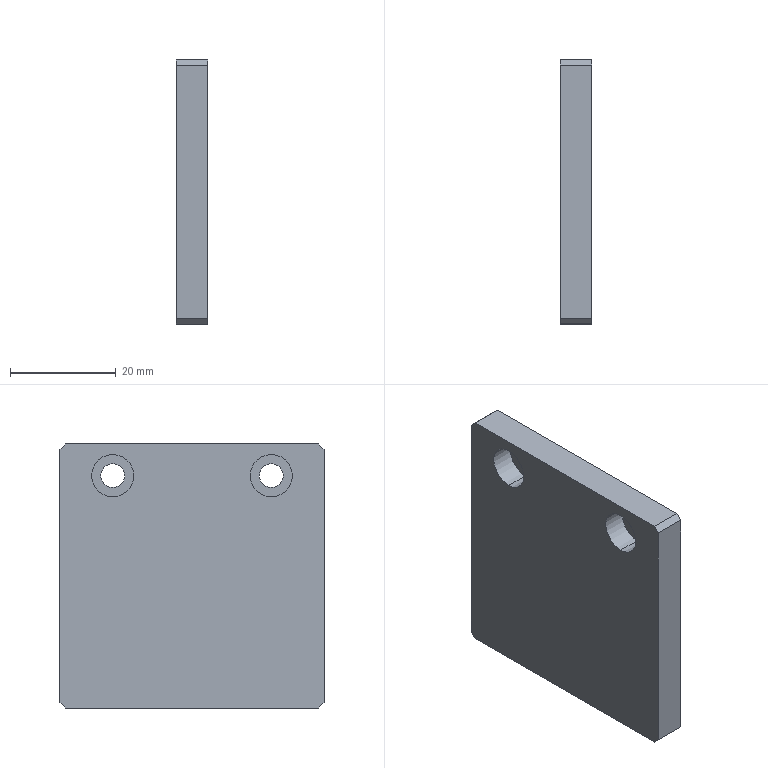Component | SolidWorks | 002MaterialPickingModuleA-1_J-008-1 | 1 solid | 20 faces | box 6 x 50 x 50 mm | volume 14495 mm3 | plane 12 | cylinder 8 | commonest cylinder face diameters 8 x4 4.5 x4 | material 45
build123d program:
from build123d import *

# Parameters (mm, degrees)
SKETCH1_W                                       = 50
SKETCH1_H                                       = 50
BOSS_EXTRUDE1_DEPTH                             = 6
M4_HEX_SOCKET_HEAD_CAP_SCREW_CBORE1_D           = 4.5
M4_HEX_SOCKET_HEAD_CAP_SCREW_CBORE1_CBORE_D     = 8
M4_HEX_SOCKET_HEAD_CAP_SCREW_CBORE1_CBORE_DEPTH = 4.4
CHAMFER1_SIZE                                   = 1


with BuildPart() as part:
    # Sketch1 → Boss-Extrude1 (new body)
    with BuildSketch(Plane(origin=(0, 0, 0), x_dir=(0, 0, -1), z_dir=(1, 0, 0))):
        Rectangle(SKETCH1_W, SKETCH1_H)
    extrude(amount=BOSS_EXTRUDE1_DEPTH)

    # M4 Hex Socket Head Cap Screw CBORE1 (through all)
    with Locations(Plane.ZY):
        with Locations((-19, 15), (-19, -15)):
            CounterBoreHole(M4_HEX_SOCKET_HEAD_CAP_SCREW_CBORE1_D / 2, M4_HEX_SOCKET_HEAD_CAP_SCREW_CBORE1_CBORE_D / 2, M4_HEX_SOCKET_HEAD_CAP_SCREW_CBORE1_CBORE_DEPTH)

    # Chamfer1
    chamfer1_edges = [part.edges().sort_by_distance(p)[0] for p in [
        (3, 25, 25),
        (3, 25, -25),
        (3, -25, -25),
        (3, -25, 25),
    ]]
    chamfer(chamfer1_edges, length=CHAMFER1_SIZE)


solid = part.part

# Placed as in the assembly
solid = solid.moved(Location((-5.675, 326.019, 403.231), (180, 0, 0)))
STEP:
#1=COLOUR_RGB('',0.7922,0.8196,0.9333);
#2=FILL_AREA_STYLE_COLOUR('',#1);
#3=FILL_AREA_STYLE('',(#2));
#4=SURFACE_STYLE_FILL_AREA(#3);
#5=SURFACE_SIDE_STYLE('',(#4));
#6=SURFACE_STYLE_USAGE(.BOTH.,#5);
#7=PRESENTATION_STYLE_ASSIGNMENT((#6));
#8=CARTESIAN_POINT('',(-0.0502,12.245,16.781));
#9=VERTEX_POINT('',#8);
#10=CARTESIAN_POINT('',(-0.0502,12.245,16.466));
#11=VERTEX_POINT('',#10);
#12=CARTESIAN_POINT('',(-0.0502,12.245,16.623));
#13=DIRECTION('',(-1.,0.,0.));
#14=DIRECTION('',(0.,0.,-1.));
#15=AXIS2_PLACEMENT_3D('',#12,#13,#14);
#16=CIRCLE('',#15,0.1575);
#17=EDGE_CURVE('',#9,#11,#16,.T.);
#18=ORIENTED_EDGE('',*,*,#17,.F.);
#19=CARTESIAN_POINT('',(-0.2234,12.245,16.781));
#20=VERTEX_POINT('',#19);
#21=CARTESIAN_POINT('',(-0.2234,12.245,16.781));
#22=DIRECTION('',(-1.,0.,0.));
#23=VECTOR('',#22,39.37);
#24=LINE('',#21,#23);
#25=EDGE_CURVE('',#9,#20,#24,.T.);
#26=ORIENTED_EDGE('',*,*,#25,.T.);
#27=CARTESIAN_POINT('',(-0.2234,12.245,16.466));
#28=VERTEX_POINT('',#27);
#29=CARTESIAN_POINT('',(-0.2234,12.245,16.623));
#30=DIRECTION('',(-1.,0.,0.));
#31=DIRECTION('',(0.,0.,-1.));
#32=AXIS2_PLACEMENT_3D('',#29,#30,#31);
#33=CIRCLE('',#32,0.1575);
#34=EDGE_CURVE('',#20,#28,#33,.T.);
#35=ORIENTED_EDGE('',*,*,#34,.T.);
#36=CARTESIAN_POINT('',(-0.2234,12.245,16.466));
#37=DIRECTION('',(-1.,0.,0.));
#38=VECTOR('',#37,39.37);
#39=LINE('',#36,#38);
#40=EDGE_CURVE('',#11,#28,#39,.T.);
#41=ORIENTED_EDGE('',*,*,#40,.F.);
#42=EDGE_LOOP('',(#18,#26,#35,#41));
#43=FACE_OUTER_BOUND('',#42,.T.);
#44=CARTESIAN_POINT('',(-0.2234,12.245,16.623));
#45=DIRECTION('',(-1.,0.,0.));
#46=DIRECTION('',(0.,0.,-1.));
#47=AXIS2_PLACEMENT_3D('',#44,#45,#46);
#48=CYLINDRICAL_SURFACE('',#47,0.1575);
#49=ADVANCED_FACE('',(#43),#48,.F.);
#50=CARTESIAN_POINT('',(0.01279,12.245,16.712));
#51=VERTEX_POINT('',#50);
#52=CARTESIAN_POINT('',(0.01279,12.245,16.535));
#53=VERTEX_POINT('',#52);
#54=CARTESIAN_POINT('',(0.01279,12.245,16.623));
#55=DIRECTION('',(-1.,0.,0.));
#56=DIRECTION('',(0.,0.,-1.));
#57=AXIS2_PLACEMENT_3D('',#54,#55,#56);
#58=CIRCLE('',#57,0.08858);
#59=EDGE_CURVE('',#51,#53,#58,.T.);
#60=ORIENTED_EDGE('',*,*,#59,.F.);
#61=CARTESIAN_POINT('',(-0.0502,12.245,16.712));
#62=VERTEX_POINT('',#61);
#63=CARTESIAN_POINT('',(-0.2234,12.245,16.712));
#64=DIRECTION('',(-1.,0.,0.));
#65=VECTOR('',#64,39.37);
#66=LINE('',#63,#65);
#67=EDGE_CURVE('',#51,#62,#66,.T.);
#68=ORIENTED_EDGE('',*,*,#67,.T.);
#69=CARTESIAN_POINT('',(-0.0502,12.245,16.535));
#70=VERTEX_POINT('',#69);
#71=CARTESIAN_POINT('',(-0.0502,12.245,16.623));
#72=DIRECTION('',(-1.,0.,0.));
#73=DIRECTION('',(0.,0.,-1.));
#74=AXIS2_PLACEMENT_3D('',#71,#72,#73);
#75=CIRCLE('',#74,0.08858);
#76=EDGE_CURVE('',#62,#70,#75,.T.);
#77=ORIENTED_EDGE('',*,*,#76,.T.);
#78=CARTESIAN_POINT('',(-0.2234,12.245,16.535));
#79=DIRECTION('',(-1.,0.,0.));
#80=VECTOR('',#79,39.37);
#81=LINE('',#78,#80);
#82=EDGE_CURVE('',#53,#70,#81,.T.);
#83=ORIENTED_EDGE('',*,*,#82,.F.);
#84=EDGE_LOOP('',(#60,#68,#77,#83));
#85=FACE_OUTER_BOUND('',#84,.T.);
#86=CARTESIAN_POINT('',(-0.2234,12.245,16.623));
#87=DIRECTION('',(-1.,0.,0.));
#88=DIRECTION('',(0.,0.,-1.));
#89=AXIS2_PLACEMENT_3D('',#86,#87,#88);
#90=CYLINDRICAL_SURFACE('',#89,0.08858);
#91=ADVANCED_FACE('',(#85),#90,.F.);
#92=CARTESIAN_POINT('',(-0.0502,13.426,16.781));
#93=VERTEX_POINT('',#92);
#94=CARTESIAN_POINT('',(-0.0502,13.426,16.466));
#95=VERTEX_POINT('',#94);
#96=CARTESIAN_POINT('',(-0.0502,13.426,16.623));
#97=DIRECTION('',(-1.,0.,0.));
#98=DIRECTION('',(0.,0.,-1.));
#99=AXIS2_PLACEMENT_3D('',#96,#97,#98);
#100=CIRCLE('',#99,0.1575);
#101=EDGE_CURVE('',#93,#95,#100,.T.);
#102=ORIENTED_EDGE('',*,*,#101,.F.);
#103=CARTESIAN_POINT('',(-0.2234,13.426,16.781));
#104=VERTEX_POINT('',#103);
#105=CARTESIAN_POINT('',(-0.2234,13.426,16.781));
#106=DIRECTION('',(-1.,0.,0.));
#107=VECTOR('',#106,39.37);
#108=LINE('',#105,#107);
#109=EDGE_CURVE('',#93,#104,#108,.T.);
#110=ORIENTED_EDGE('',*,*,#109,.T.);
#111=CARTESIAN_POINT('',(-0.2234,13.426,16.466));
#112=VERTEX_POINT('',#111);
#113=CARTESIAN_POINT('',(-0.2234,13.426,16.623));
#114=DIRECTION('',(-1.,0.,0.));
#115=DIRECTION('',(0.,0.,-1.));
#116=AXIS2_PLACEMENT_3D('',#113,#114,#115);
#117=CIRCLE('',#116,0.1575);
#118=EDGE_CURVE('',#104,#112,#117,.T.);
#119=ORIENTED_EDGE('',*,*,#118,.T.);
#120=CARTESIAN_POINT('',(-0.2234,13.426,16.466));
#121=DIRECTION('',(-1.,0.,0.));
#122=VECTOR('',#121,39.37);
#123=LINE('',#120,#122);
#124=EDGE_CURVE('',#95,#112,#123,.T.);
#125=ORIENTED_EDGE('',*,*,#124,.F.);
#126=EDGE_LOOP('',(#102,#110,#119,#125));
#127=FACE_OUTER_BOUND('',#126,.T.);
#128=CARTESIAN_POINT('',(-0.2234,13.426,16.623));
#129=DIRECTION('',(-1.,0.,0.));
#130=DIRECTION('',(0.,0.,-1.));
#131=AXIS2_PLACEMENT_3D('',#128,#129,#130);
#132=CYLINDRICAL_SURFACE('',#131,0.1575);
#133=ADVANCED_FACE('',(#127),#132,.F.);
#134=CARTESIAN_POINT('',(0.01279,13.426,16.712));
#135=VERTEX_POINT('',#134);
#136=CARTESIAN_POINT('',(0.01279,13.426,16.535));
#137=VERTEX_POINT('',#136);
#138=CARTESIAN_POINT('',(0.01279,13.426,16.623));
#139=DIRECTION('',(-1.,0.,0.));
#140=DIRECTION('',(0.,0.,-1.));
#141=AXIS2_PLACEMENT_3D('',#138,#139,#140);
#142=CIRCLE('',#141,0.08858);
#143=EDGE_CURVE('',#135,#137,#142,.T.);
#144=ORIENTED_EDGE('',*,*,#143,.F.);
#145=CARTESIAN_POINT('',(-0.0502,13.426,16.712));
#146=VERTEX_POINT('',#145);
#147=CARTESIAN_POINT('',(-0.2234,13.426,16.712));
#148=DIRECTION('',(-1.,0.,0.));
#149=VECTOR('',#148,39.37);
#150=LINE('',#147,#149);
#151=EDGE_CURVE('',#135,#146,#150,.T.);
#152=ORIENTED_EDGE('',*,*,#151,.T.);
#153=CARTESIAN_POINT('',(-0.0502,13.426,16.535));
#154=VERTEX_POINT('',#153);
#155=CARTESIAN_POINT('',(-0.0502,13.426,16.623));
#156=DIRECTION('',(-1.,0.,0.));
#157=DIRECTION('',(0.,0.,-1.));
#158=AXIS2_PLACEMENT_3D('',#155,#156,#157);
#159=CIRCLE('',#158,0.08858);
#160=EDGE_CURVE('',#146,#154,#159,.T.);
#161=ORIENTED_EDGE('',*,*,#160,.T.);
#162=CARTESIAN_POINT('',(-0.2234,13.426,16.535));
#163=DIRECTION('',(-1.,0.,0.));
#164=VECTOR('',#163,39.37);
#165=LINE('',#162,#164);
#166=EDGE_CURVE('',#137,#154,#165,.T.);
#167=ORIENTED_EDGE('',*,*,#166,.F.);
#168=EDGE_LOOP('',(#144,#152,#161,#167));
#169=FACE_OUTER_BOUND('',#168,.T.);
#170=CARTESIAN_POINT('',(-0.2234,13.426,16.623));
#171=DIRECTION('',(-1.,0.,0.));
#172=DIRECTION('',(0.,0.,-1.));
#173=AXIS2_PLACEMENT_3D('',#170,#171,#172);
#174=CYLINDRICAL_SURFACE('',#173,0.08858);
#175=ADVANCED_FACE('',(#169),#174,.F.);
#176=CARTESIAN_POINT('',(-0.2234,11.89,14.891));
#177=VERTEX_POINT('',#176);
#178=CARTESIAN_POINT('',(-0.2234,13.78,14.891));
#179=VERTEX_POINT('',#178);
#180=CARTESIAN_POINT('',(-0.2234,13.82,14.891));
#181=DIRECTION('',(0.,1.,0.));
#182=VECTOR('',#181,39.37);
#183=LINE('',#180,#182);
#184=EDGE_CURVE('',#177,#179,#183,.T.);
#185=ORIENTED_EDGE('',*,*,#184,.T.);
#186=CARTESIAN_POINT('',(0.01279,13.78,14.891));
#187=VERTEX_POINT('',#186);
#188=CARTESIAN_POINT('',(0.01279,13.78,14.891));
#189=DIRECTION('',(1.,-0.,0.));
#190=VECTOR('',#189,39.37);
#191=LINE('',#188,#190);
#192=EDGE_CURVE('',#179,#187,#191,.T.);
#193=ORIENTED_EDGE('',*,*,#192,.T.);
#194=CARTESIAN_POINT('',(0.01279,11.89,14.891));
#195=VERTEX_POINT('',#194);
#196=CARTESIAN_POINT('',(0.01279,13.82,14.891));
#197=DIRECTION('',(0.,1.,0.));
#198=VECTOR('',#197,39.37);
#199=LINE('',#196,#198);
#200=EDGE_CURVE('',#195,#187,#199,.T.);
#201=ORIENTED_EDGE('',*,*,#200,.F.);
#202=CARTESIAN_POINT('',(0.01279,11.89,14.891));
#203=DIRECTION('',(-1.,0.,0.));
#204=VECTOR('',#203,39.37);
#205=LINE('',#202,#204);
#206=EDGE_CURVE('',#195,#177,#205,.T.);
#207=ORIENTED_EDGE('',*,*,#206,.T.);
#208=EDGE_LOOP('',(#185,#193,#201,#207));
#209=FACE_OUTER_BOUND('',#208,.T.);
#210=CARTESIAN_POINT('',(0.01279,13.82,14.891));
#211=DIRECTION('',(0.,0.,1.));
#212=DIRECTION('',(-1.,0.,0.));
#213=AXIS2_PLACEMENT_3D('',#210,#211,#212);
#214=PLANE('',#213);
#215=ADVANCED_FACE('',(#209),#214,.F.);
#216=CARTESIAN_POINT('',(0.01279,13.82,14.93));
#217=VERTEX_POINT('',#216);
#218=CARTESIAN_POINT('',(0.01279,13.82,16.82));
#219=VERTEX_POINT('',#218);
#220=CARTESIAN_POINT('',(0.01279,13.82,16.859));
#221=DIRECTION('',(-0.,-0.,1.));
#222=VECTOR('',#221,39.37);
#223=LINE('',#220,#222);
#224=EDGE_CURVE('',#217,#219,#223,.T.);
#225=ORIENTED_EDGE('',*,*,#224,.F.);
#226=CARTESIAN_POINT('',(-0.2234,13.82,14.93));
#227=VERTEX_POINT('',#226);
#228=CARTESIAN_POINT('',(0.01279,13.82,14.93));
#229=DIRECTION('',(-1.,0.,0.));
#230=VECTOR('',#229,39.37);
#231=LINE('',#228,#230);
#232=EDGE_CURVE('',#217,#227,#231,.T.);
#233=ORIENTED_EDGE('',*,*,#232,.T.);
#234=CARTESIAN_POINT('',(-0.2234,13.82,16.82));
#235=VERTEX_POINT('',#234);
#236=CARTESIAN_POINT('',(-0.2234,13.82,16.859));
#237=DIRECTION('',(-0.,-0.,1.));
#238=VECTOR('',#237,39.37);
#239=LINE('',#236,#238);
#240=EDGE_CURVE('',#227,#235,#239,.T.);
#241=ORIENTED_EDGE('',*,*,#240,.T.);
#242=CARTESIAN_POINT('',(0.01279,13.82,16.82));
#243=DIRECTION('',(1.,-0.,0.));
#244=VECTOR('',#243,39.37);
#245=LINE('',#242,#244);
#246=EDGE_CURVE('',#235,#219,#245,.T.);
#247=ORIENTED_EDGE('',*,*,#246,.T.);
#248=EDGE_LOOP('',(#225,#233,#241,#247));
#249=FACE_OUTER_BOUND('',#248,.T.);
#250=CARTESIAN_POINT('',(0.01279,13.82,16.859));
#251=DIRECTION('',(-0.,-1.,-0.));
#252=DIRECTION('',(0.,0.,-1.));
#253=AXIS2_PLACEMENT_3D('',#250,#251,#252);
#254=PLANE('',#253);
#255=ADVANCED_FACE('',(#249),#254,.F.);
#256=CARTESIAN_POINT('',(0.01279,13.78,16.859));
#257=VERTEX_POINT('',#256);
#258=CARTESIAN_POINT('',(0.01279,11.89,16.859));
#259=VERTEX_POINT('',#258);
#260=CARTESIAN_POINT('',(0.01279,13.82,16.859));
#261=DIRECTION('',(-0.,-1.,0.));
#262=VECTOR('',#261,39.37);
#263=LINE('',#260,#262);
#264=EDGE_CURVE('',#257,#259,#263,.T.);
#265=ORIENTED_EDGE('',*,*,#264,.F.);
#266=CARTESIAN_POINT('',(-0.2234,13.78,16.859));
#267=VERTEX_POINT('',#266);
#268=CARTESIAN_POINT('',(0.01279,13.78,16.859));
#269=DIRECTION('',(-1.,0.,0.));
#270=VECTOR('',#269,39.37);
#271=LINE('',#268,#270);
#272=EDGE_CURVE('',#257,#267,#271,.T.);
#273=ORIENTED_EDGE('',*,*,#272,.T.);
#274=CARTESIAN_POINT('',(-0.2234,11.89,16.859));
#275=VERTEX_POINT('',#274);
#276=CARTESIAN_POINT('',(-0.2234,13.82,16.859));
#277=DIRECTION('',(-0.,-1.,0.));
#278=VECTOR('',#277,39.37);
#279=LINE('',#276,#278);
#280=EDGE_CURVE('',#267,#275,#279,.T.);
#281=ORIENTED_EDGE('',*,*,#280,.T.);
#282=CARTESIAN_POINT('',(0.01279,11.89,16.859));
#283=DIRECTION('',(1.,-0.,0.));
#284=VECTOR('',#283,39.37);
#285=LINE('',#282,#284);
#286=EDGE_CURVE('',#275,#259,#285,.T.);
#287=ORIENTED_EDGE('',*,*,#286,.T.);
#288=EDGE_LOOP('',(#265,#273,#281,#287));
#289=FACE_OUTER_BOUND('',#288,.T.);
#290=CARTESIAN_POINT('',(0.01279,13.82,16.859));
#291=DIRECTION('',(0.,0.,-1.));
#292=DIRECTION('',(1.,-0.,0.));
#293=AXIS2_PLACEMENT_3D('',#290,#291,#292);
#294=PLANE('',#293);
#295=ADVANCED_FACE('',(#289),#294,.F.);
#296=CARTESIAN_POINT('',(-0.2234,11.851,16.82));
#297=VERTEX_POINT('',#296);
#298=CARTESIAN_POINT('',(-0.2234,11.851,14.93));
#299=VERTEX_POINT('',#298);
#300=CARTESIAN_POINT('',(-0.2234,11.851,16.859));
#301=DIRECTION('',(0.,0.,-1.));
#302=VECTOR('',#301,39.37);
#303=LINE('',#300,#302);
#304=EDGE_CURVE('',#297,#299,#303,.T.);
#305=ORIENTED_EDGE('',*,*,#304,.T.);
#306=CARTESIAN_POINT('',(0.01279,11.851,14.93));
#307=VERTEX_POINT('',#306);
#308=CARTESIAN_POINT('',(0.01279,11.851,14.93));
#309=DIRECTION('',(1.,-0.,0.));
#310=VECTOR('',#309,39.37);
#311=LINE('',#308,#310);
#312=EDGE_CURVE('',#299,#307,#311,.T.);
#313=ORIENTED_EDGE('',*,*,#312,.T.);
#314=CARTESIAN_POINT('',(0.01279,11.851,16.82));
#315=VERTEX_POINT('',#314);
#316=CARTESIAN_POINT('',(0.01279,11.851,16.859));
#317=DIRECTION('',(0.,0.,-1.));
#318=VECTOR('',#317,39.37);
#319=LINE('',#316,#318);
#320=EDGE_CURVE('',#315,#307,#319,.T.);
#321=ORIENTED_EDGE('',*,*,#320,.F.);
#322=CARTESIAN_POINT('',(0.01279,11.851,16.82));
#323=DIRECTION('',(-1.,0.,0.));
#324=VECTOR('',#323,39.37);
#325=LINE('',#322,#324);
#326=EDGE_CURVE('',#315,#297,#325,.T.);
#327=ORIENTED_EDGE('',*,*,#326,.T.);
#328=EDGE_LOOP('',(#305,#313,#321,#327));
#329=FACE_OUTER_BOUND('',#328,.T.);
#330=CARTESIAN_POINT('',(0.01279,11.851,16.859));
#331=DIRECTION('',(0.,1.,0.));
#332=DIRECTION('',(-0.,-0.,1.));
#333=AXIS2_PLACEMENT_3D('',#330,#331,#332);
#334=PLANE('',#333);
#335=ADVANCED_FACE('',(#329),#334,.F.);
#336=CARTESIAN_POINT('',(0.01279,12.245,16.623));
#337=DIRECTION('',(-1.,0.,0.));
#338=DIRECTION('',(0.,0.,-1.));
#339=AXIS2_PLACEMENT_3D('',#336,#337,#338);
#340=CIRCLE('',#339,0.08858);
#341=EDGE_CURVE('',#53,#51,#340,.T.);
#342=ORIENTED_EDGE('',*,*,#341,.T.);
#343=ORIENTED_EDGE('',*,*,#59,.T.);
#344=EDGE_LOOP('',(#342,#343));
#345=FACE_BOUND('',#344,.T.);
#346=CARTESIAN_POINT('',(0.01279,13.426,16.623));
#347=DIRECTION('',(-1.,0.,0.));
#348=DIRECTION('',(0.,0.,-1.));
#349=AXIS2_PLACEMENT_3D('',#346,#347,#348);
#350=CIRCLE('',#349,0.08858);
#351=EDGE_CURVE('',#137,#135,#350,.T.);
#352=ORIENTED_EDGE('',*,*,#351,.T.);
#353=ORIENTED_EDGE('',*,*,#143,.T.);
#354=EDGE_LOOP('',(#352,#353));
#355=FACE_BOUND('',#354,.T.);
#356=ORIENTED_EDGE('',*,*,#200,.T.);
#357=CARTESIAN_POINT('',(0.01279,13.8,14.911));
#358=DIRECTION('',(0.,0.7071,0.7071));
#359=VECTOR('',#358,39.37);
#360=LINE('',#357,#359);
#361=EDGE_CURVE('',#187,#217,#360,.T.);
#362=ORIENTED_EDGE('',*,*,#361,.T.);
#363=ORIENTED_EDGE('',*,*,#224,.T.);
#364=CARTESIAN_POINT('',(0.01279,13.8,16.84));
#365=DIRECTION('',(-0.,-0.7071,0.7071));
#366=VECTOR('',#365,39.37);
#367=LINE('',#364,#366);
#368=EDGE_CURVE('',#219,#257,#367,.T.);
#369=ORIENTED_EDGE('',*,*,#368,.T.);
#370=ORIENTED_EDGE('',*,*,#264,.T.);
#371=CARTESIAN_POINT('',(0.01279,11.871,16.84));
#372=DIRECTION('',(-0.,-0.7071,-0.7071));
#373=VECTOR('',#372,39.37);
#374=LINE('',#371,#373);
#375=EDGE_CURVE('',#259,#315,#374,.T.);
#376=ORIENTED_EDGE('',*,*,#375,.T.);
#377=ORIENTED_EDGE('',*,*,#320,.T.);
#378=CARTESIAN_POINT('',(0.01279,11.871,14.911));
#379=DIRECTION('',(0.,0.7071,-0.7071));
#380=VECTOR('',#379,39.37);
#381=LINE('',#378,#380);
#382=EDGE_CURVE('',#307,#195,#381,.T.);
#383=ORIENTED_EDGE('',*,*,#382,.T.);
#384=EDGE_LOOP('',(#356,#362,#363,#369,#370,#376,#377,#383));
#385=FACE_OUTER_BOUND('',#384,.T.);
#386=CARTESIAN_POINT('',(0.01279,12.835,15.875));
#387=DIRECTION('',(1.,-0.,0.));
#388=DIRECTION('',(0.,0.,1.));
#389=AXIS2_PLACEMENT_3D('',#386,#387,#388);
#390=PLANE('',#389);
#391=ADVANCED_FACE('',(#345,#355,#385),#390,.T.);
#392=CARTESIAN_POINT('',(-0.2234,12.245,16.623));
#393=DIRECTION('',(-1.,0.,0.));
#394=DIRECTION('',(0.,0.,-1.));
#395=AXIS2_PLACEMENT_3D('',#392,#393,#394);
#396=CIRCLE('',#395,0.1575);
#397=EDGE_CURVE('',#28,#20,#396,.T.);
#398=ORIENTED_EDGE('',*,*,#397,.F.);
#399=ORIENTED_EDGE('',*,*,#34,.F.);
#400=EDGE_LOOP('',(#398,#399));
#401=FACE_BOUND('',#400,.T.);
#402=CARTESIAN_POINT('',(-0.2234,13.426,16.623));
#403=DIRECTION('',(-1.,0.,0.));
#404=DIRECTION('',(0.,0.,-1.));
#405=AXIS2_PLACEMENT_3D('',#402,#403,#404);
#406=CIRCLE('',#405,0.1575);
#407=EDGE_CURVE('',#112,#104,#406,.T.);
#408=ORIENTED_EDGE('',*,*,#407,.F.);
#409=ORIENTED_EDGE('',*,*,#118,.F.);
#410=EDGE_LOOP('',(#408,#409));
#411=FACE_BOUND('',#410,.T.);
#412=ORIENTED_EDGE('',*,*,#240,.F.);
#413=CARTESIAN_POINT('',(-0.2234,13.82,14.93));
#414=DIRECTION('',(-0.,-0.7071,-0.7071));
#415=VECTOR('',#414,39.37);
#416=LINE('',#413,#415);
#417=EDGE_CURVE('',#227,#179,#416,.T.);
#418=ORIENTED_EDGE('',*,*,#417,.T.);
#419=ORIENTED_EDGE('',*,*,#184,.F.);
#420=CARTESIAN_POINT('',(-0.2234,11.89,14.891));
#421=DIRECTION('',(-0.,-0.7071,0.7071));
#422=VECTOR('',#421,39.37);
#423=LINE('',#420,#422);
#424=EDGE_CURVE('',#177,#299,#423,.T.);
#425=ORIENTED_EDGE('',*,*,#424,.T.);
#426=ORIENTED_EDGE('',*,*,#304,.F.);
#427=CARTESIAN_POINT('',(-0.2234,11.851,16.82));
#428=DIRECTION('',(0.,0.7071,0.7071));
#429=VECTOR('',#428,39.37);
#430=LINE('',#427,#429);
#431=EDGE_CURVE('',#297,#275,#430,.T.);
#432=ORIENTED_EDGE('',*,*,#431,.T.);
#433=ORIENTED_EDGE('',*,*,#280,.F.);
#434=CARTESIAN_POINT('',(-0.2234,13.78,16.859));
#435=DIRECTION('',(0.,0.7071,-0.7071));
#436=VECTOR('',#435,39.37);
#437=LINE('',#434,#436);
#438=EDGE_CURVE('',#267,#235,#437,.T.);
#439=ORIENTED_EDGE('',*,*,#438,.T.);
#440=EDGE_LOOP('',(#412,#418,#419,#425,#426,#432,#433,#439));
#441=FACE_OUTER_BOUND('',#440,.T.);
#442=CARTESIAN_POINT('',(-0.2234,12.835,15.875));
#443=DIRECTION('',(1.,-0.,0.));
#444=DIRECTION('',(0.,0.,1.));
#445=AXIS2_PLACEMENT_3D('',#442,#443,#444);
#446=PLANE('',#445);
#447=ADVANCED_FACE('',(#401,#411,#441),#446,.F.);
#448=ORIENTED_EDGE('',*,*,#151,.F.);
#449=ORIENTED_EDGE('',*,*,#351,.F.);
#450=ORIENTED_EDGE('',*,*,#166,.T.);
#451=CARTESIAN_POINT('',(-0.0502,13.426,16.623));
#452=DIRECTION('',(-1.,0.,0.));
#453=DIRECTION('',(0.,0.,-1.));
#454=AXIS2_PLACEMENT_3D('',#451,#452,#453);
#455=CIRCLE('',#454,0.08858);
#456=EDGE_CURVE('',#154,#146,#455,.T.);
#457=ORIENTED_EDGE('',*,*,#456,.T.);
#458=EDGE_LOOP('',(#448,#449,#450,#457));
#459=FACE_OUTER_BOUND('',#458,.T.);
#460=CARTESIAN_POINT('',(-0.2234,13.426,16.623));
#461=DIRECTION('',(-1.,0.,0.));
#462=DIRECTION('',(0.,0.,-1.));
#463=AXIS2_PLACEMENT_3D('',#460,#461,#462);
#464=CYLINDRICAL_SURFACE('',#463,0.08858);
#465=ADVANCED_FACE('',(#459),#464,.F.);
#466=ORIENTED_EDGE('',*,*,#456,.F.);
#467=ORIENTED_EDGE('',*,*,#160,.F.);
#468=EDGE_LOOP('',(#466,#467));
#469=FACE_BOUND('',#468,.T.);
#470=CARTESIAN_POINT('',(-0.0502,13.426,16.623));
#471=DIRECTION('',(-1.,0.,0.));
#472=DIRECTION('',(0.,0.,-1.));
#473=AXIS2_PLACEMENT_3D('',#470,#471,#472);
#474=CIRCLE('',#473,0.1575);
#475=EDGE_CURVE('',#95,#93,#474,.T.);
#476=ORIENTED_EDGE('',*,*,#475,.T.);
#477=ORIENTED_EDGE('',*,*,#101,.T.);
#478=EDGE_LOOP('',(#476,#477));
#479=FACE_OUTER_BOUND('',#478,.T.);
#480=CARTESIAN_POINT('',(-0.0502,13.337,16.623));
#481=DIRECTION('',(1.,-0.,0.));
#482=DIRECTION('',(0.,0.,1.));
#483=AXIS2_PLACEMENT_3D('',#480,#481,#482);
#484=PLANE('',#483);
#485=ADVANCED_FACE('',(#469,#479),#484,.F.);
#486=ORIENTED_EDGE('',*,*,#109,.F.);
#487=ORIENTED_EDGE('',*,*,#475,.F.);
#488=ORIENTED_EDGE('',*,*,#124,.T.);
#489=ORIENTED_EDGE('',*,*,#407,.T.);
#490=EDGE_LOOP('',(#486,#487,#488,#489));
#491=FACE_OUTER_BOUND('',#490,.T.);
#492=CARTESIAN_POINT('',(-0.2234,13.426,16.623));
#493=DIRECTION('',(-1.,0.,0.));
#494=DIRECTION('',(0.,0.,-1.));
#495=AXIS2_PLACEMENT_3D('',#492,#493,#494);
#496=CYLINDRICAL_SURFACE('',#495,0.1575);
#497=ADVANCED_FACE('',(#491),#496,.F.);
#498=ORIENTED_EDGE('',*,*,#67,.F.);
#499=ORIENTED_EDGE('',*,*,#341,.F.);
#500=ORIENTED_EDGE('',*,*,#82,.T.);
#501=CARTESIAN_POINT('',(-0.0502,12.245,16.623));
#502=DIRECTION('',(-1.,0.,0.));
#503=DIRECTION('',(0.,0.,-1.));
#504=AXIS2_PLACEMENT_3D('',#501,#502,#503);
#505=CIRCLE('',#504,0.08858);
#506=EDGE_CURVE('',#70,#62,#505,.T.);
#507=ORIENTED_EDGE('',*,*,#506,.T.);
#508=EDGE_LOOP('',(#498,#499,#500,#507));
#509=FACE_OUTER_BOUND('',#508,.T.);
#510=CARTESIAN_POINT('',(-0.2234,12.245,16.623));
#511=DIRECTION('',(-1.,0.,0.));
#512=DIRECTION('',(0.,0.,-1.));
#513=AXIS2_PLACEMENT_3D('',#510,#511,#512);
#514=CYLINDRICAL_SURFACE('',#513,0.08858);
#515=ADVANCED_FACE('',(#509),#514,.F.);
#516=ORIENTED_EDGE('',*,*,#506,.F.);
#517=ORIENTED_EDGE('',*,*,#76,.F.);
#518=EDGE_LOOP('',(#516,#517));
#519=FACE_BOUND('',#518,.T.);
#520=CARTESIAN_POINT('',(-0.0502,12.245,16.623));
#521=DIRECTION('',(-1.,0.,0.));
#522=DIRECTION('',(0.,0.,-1.));
#523=AXIS2_PLACEMENT_3D('',#520,#521,#522);
#524=CIRCLE('',#523,0.1575);
#525=EDGE_CURVE('',#11,#9,#524,.T.);
#526=ORIENTED_EDGE('',*,*,#525,.T.);
#527=ORIENTED_EDGE('',*,*,#17,.T.);
#528=EDGE_LOOP('',(#526,#527));
#529=FACE_OUTER_BOUND('',#528,.T.);
#530=CARTESIAN_POINT('',(-0.0502,12.156,16.623));
#531=DIRECTION('',(1.,-0.,0.));
#532=DIRECTION('',(0.,0.,1.));
#533=AXIS2_PLACEMENT_3D('',#530,#531,#532);
#534=PLANE('',#533);
#535=ADVANCED_FACE('',(#519,#529),#534,.F.);
#536=ORIENTED_EDGE('',*,*,#25,.F.);
#537=ORIENTED_EDGE('',*,*,#525,.F.);
#538=ORIENTED_EDGE('',*,*,#40,.T.);
#539=ORIENTED_EDGE('',*,*,#397,.T.);
#540=EDGE_LOOP('',(#536,#537,#538,#539));
#541=FACE_OUTER_BOUND('',#540,.T.);
#542=CARTESIAN_POINT('',(-0.2234,12.245,16.623));
#543=DIRECTION('',(-1.,0.,0.));
#544=DIRECTION('',(0.,0.,-1.));
#545=AXIS2_PLACEMENT_3D('',#542,#543,#544);
#546=CYLINDRICAL_SURFACE('',#545,0.1575);
#547=ADVANCED_FACE('',(#541),#546,.F.);
#548=ORIENTED_EDGE('',*,*,#361,.F.);
#549=ORIENTED_EDGE('',*,*,#192,.F.);
#550=ORIENTED_EDGE('',*,*,#417,.F.);
#551=ORIENTED_EDGE('',*,*,#232,.F.);
#552=EDGE_LOOP('',(#548,#549,#550,#551));
#553=FACE_OUTER_BOUND('',#552,.T.);
#554=CARTESIAN_POINT('',(0.01279,13.82,14.93));
#555=DIRECTION('',(-0.,-0.7071,0.7071));
#556=DIRECTION('',(-1.,0.,0.));
#557=AXIS2_PLACEMENT_3D('',#554,#555,#556);
#558=PLANE('',#557);
#559=ADVANCED_FACE('',(#553),#558,.F.);
#560=ORIENTED_EDGE('',*,*,#382,.F.);
#561=ORIENTED_EDGE('',*,*,#312,.F.);
#562=ORIENTED_EDGE('',*,*,#424,.F.);
#563=ORIENTED_EDGE('',*,*,#206,.F.);
#564=EDGE_LOOP('',(#560,#561,#562,#563));
#565=FACE_OUTER_BOUND('',#564,.T.);
#566=CARTESIAN_POINT('',(0.01279,11.89,14.891));
#567=DIRECTION('',(0.,0.7071,0.7071));
#568=DIRECTION('',(-1.,0.,0.));
#569=AXIS2_PLACEMENT_3D('',#566,#567,#568);
#570=PLANE('',#569);
#571=ADVANCED_FACE('',(#565),#570,.F.);
#572=ORIENTED_EDGE('',*,*,#368,.F.);
#573=ORIENTED_EDGE('',*,*,#246,.F.);
#574=ORIENTED_EDGE('',*,*,#438,.F.);
#575=ORIENTED_EDGE('',*,*,#272,.F.);
#576=EDGE_LOOP('',(#572,#573,#574,#575));
#577=FACE_OUTER_BOUND('',#576,.T.);
#578=CARTESIAN_POINT('',(0.01279,13.78,16.859));
#579=DIRECTION('',(-0.,-0.7071,-0.7071));
#580=DIRECTION('',(-1.,0.,0.));
#581=AXIS2_PLACEMENT_3D('',#578,#579,#580);
#582=PLANE('',#581);
#583=ADVANCED_FACE('',(#577),#582,.F.);
#584=ORIENTED_EDGE('',*,*,#375,.F.);
#585=ORIENTED_EDGE('',*,*,#286,.F.);
#586=ORIENTED_EDGE('',*,*,#431,.F.);
#587=ORIENTED_EDGE('',*,*,#326,.F.);
#588=EDGE_LOOP('',(#584,#585,#586,#587));
#589=FACE_OUTER_BOUND('',#588,.T.);
#590=CARTESIAN_POINT('',(0.01279,11.851,16.82));
#591=DIRECTION('',(0.,0.7071,-0.7071));
#592=DIRECTION('',(-1.,0.,0.));
#593=AXIS2_PLACEMENT_3D('',#590,#591,#592);
#594=PLANE('',#593);
#595=ADVANCED_FACE('',(#589),#594,.F.);
#596=CLOSED_SHELL('',(#49,#91,#133,#175,#215,#255,#295,#335,#391,#447,#465,#485,#497,#515,#535,#547,#559,#571,#583,#595));
#597=MANIFOLD_SOLID_BREP('',#596);
#598=STYLED_ITEM('',(#7),#597);
#599=(LENGTH_UNIT()NAMED_UNIT(*)SI_UNIT($,.METRE.));
#600=LENGTH_MEASURE_WITH_UNIT(LENGTH_MEASURE(0.0254),#599);
#601=DIMENSIONAL_EXPONENTS(1.,0.,0.,0.,0.,0.,0.);
#602=(CONVERSION_BASED_UNIT('',#600)LENGTH_UNIT()NAMED_UNIT(#601));
#603=UNCERTAINTY_MEASURE_WITH_UNIT(LENGTH_MEASURE(0.00001),#602,'','');
#604=(NAMED_UNIT(*)PLANE_ANGLE_UNIT()SI_UNIT($,.RADIAN.));
#605=(NAMED_UNIT(*)SI_UNIT($,.STERADIAN.)SOLID_ANGLE_UNIT());
#606=(GEOMETRIC_REPRESENTATION_CONTEXT(3)GLOBAL_UNCERTAINTY_ASSIGNED_CONTEXT((#603))GLOBAL_UNIT_ASSIGNED_CONTEXT((#602,#604,#605))REPRESENTATION_CONTEXT('',''));
#607=MECHANICAL_DESIGN_GEOMETRIC_PRESENTATION_REPRESENTATION('',(#598),#606);
#608=PRESENTATION_LAYER_ASSIGNMENT('','',(#598));
#609=CARTESIAN_POINT('',(0.,0.,0.));
#610=DIRECTION('',(0.,0.,1.));
#611=DIRECTION('',(1.,0.,0.));
#612=AXIS2_PLACEMENT_3D('',#609,#610,#611);
#613=(LENGTH_UNIT()NAMED_UNIT(*)SI_UNIT($,.METRE.));
#614=LENGTH_MEASURE_WITH_UNIT(LENGTH_MEASURE(0.0254),#613);
#615=DIMENSIONAL_EXPONENTS(1.,0.,0.,0.,0.,0.,0.);
#616=(CONVERSION_BASED_UNIT('',#614)LENGTH_UNIT()NAMED_UNIT(#615));
#617=UNCERTAINTY_MEASURE_WITH_UNIT(LENGTH_MEASURE(0.00001),#616,'','');
#618=(NAMED_UNIT(*)PLANE_ANGLE_UNIT()SI_UNIT($,.RADIAN.));
#619=(NAMED_UNIT(*)SI_UNIT($,.STERADIAN.)SOLID_ANGLE_UNIT());
#620=(GEOMETRIC_REPRESENTATION_CONTEXT(3)GLOBAL_UNCERTAINTY_ASSIGNED_CONTEXT((#617))GLOBAL_UNIT_ASSIGNED_CONTEXT((#616,#618,#619))REPRESENTATION_CONTEXT('',''));
#621=ADVANCED_BREP_SHAPE_REPRESENTATION('',(#597,#612),#620);